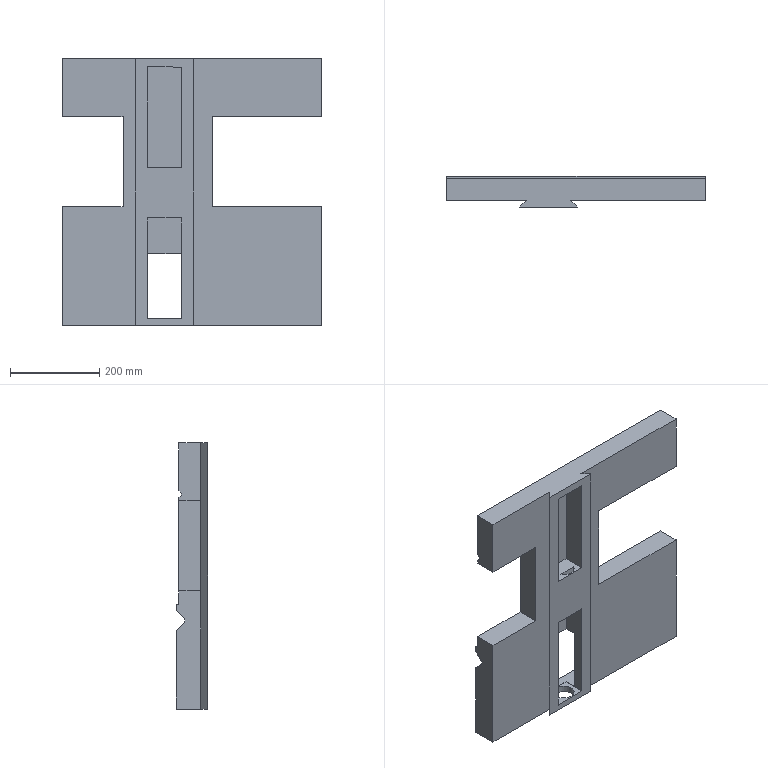Component | NX | LARGE_BASE | 1 solid | 49 faces | volume 10408821 mm3 | plane 47 | cylinder 2 | commonest cylinder face diameters 45 x2